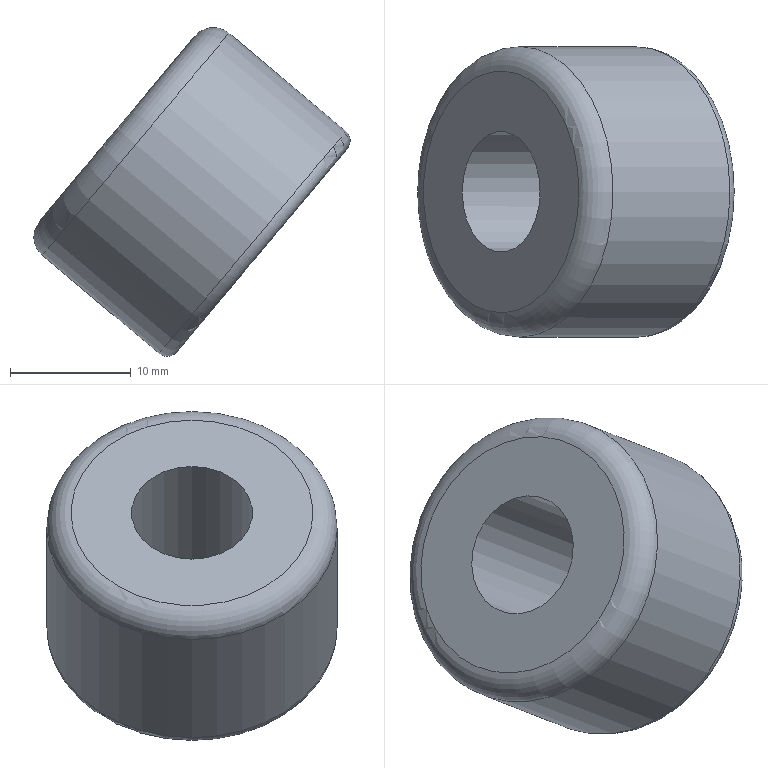Component | NX | BASEBUSHING1_2 | 1 solid | 6 faces | box 26.17 x 24 x 27.2 mm | volume 5761 mm3 | cylinder 2 | plane 2 | torus 2 | commonest cylinder face diameters 24 x1 10 x1
STEP:
#1=CARTESIAN_POINT('',(0.,0.,0.));
#2=DIRECTION('',(0.,0.,1.));
#3=DIRECTION('',(1.,0.,0.));
#4=AXIS2_PLACEMENT_3D('',#1,#2,#3);
#5=CARTESIAN_POINT('',(429.187,0.,-30.182));
#6=VERTEX_POINT('',#5);
#7=CARTESIAN_POINT('',(421.473,0.,-39.375));
#8=DIRECTION('',(0.766,0.,-0.6428));
#9=DIRECTION('',(0.6428,0.,0.766));
#10=AXIS2_PLACEMENT_3D('',#7,#8,#9);
#11=CIRCLE('',#10,12.);
#12=CARTESIAN_POINT('',(431.907,0.,-48.13));
#13=DIRECTION('',(-0.766,0.,0.6428));
#14=DIRECTION('',(0.6428,0.,0.766));
#15=AXIS2_PLACEMENT_3D('',#12,#13,#14);
#16=CYLINDRICAL_SURFACE('',#15,12.);
#17=CARTESIAN_POINT('',(6.283,13.62));
#18=DIRECTION('',(-1.,0.));
#19=VECTOR('',#18,1.);
#20=LINE('',#17,#19);
#21=(GEOMETRIC_REPRESENTATION_CONTEXT(2)PARAMETRIC_REPRESENTATION_CONTEXT()REPRESENTATION_CONTEXT('',''));
#22=DEFINITIONAL_REPRESENTATION('',(#20),#21);
#23=PCURVE('',#16,#22);
#24=CARTESIAN_POINT('',(421.473,0.,-39.375));
#25=DIRECTION('',(-0.766,0.,0.6428));
#26=DIRECTION('',(0.6428,0.,0.766));
#27=AXIS2_PLACEMENT_3D('',#24,#25,#26);
#28=TOROIDAL_SURFACE('',#27,10.,2.);
#29=CARTESIAN_POINT('',(6.283,6.283));
#30=DIRECTION('',(-1.,0.));
#31=VECTOR('',#30,1.);
#32=LINE('',#29,#31);
#33=(GEOMETRIC_REPRESENTATION_CONTEXT(2)PARAMETRIC_REPRESENTATION_CONTEXT()REPRESENTATION_CONTEXT('',''));
#34=DEFINITIONAL_REPRESENTATION('',(#32),#33);
#35=PCURVE('',#28,#34);
#36=SURFACE_CURVE('',#11,(#23,#35),.PCURVE_S1.);
#37=EDGE_CURVE('',#6,#6,#36,.T.);
#38=ORIENTED_EDGE('',*,*,#37,.T.);
#39=CARTESIAN_POINT('',(438.854,0.,-38.295));
#40=VERTEX_POINT('',#39);
#41=CARTESIAN_POINT('',(438.854,-0.,-38.295));
#42=CARTESIAN_POINT('',(429.187,-0.,-30.182));
#43=B_SPLINE_CURVE_WITH_KNOTS('',1,(#41,#42),.UNSPECIFIED.,.F.,.F.,(2,2),(1.,13.62),.PIECEWISE_BEZIER_KNOTS.);
#44=CARTESIAN_POINT('',(0.,0.));
#45=DIRECTION('',(0.,1.));
#46=VECTOR('',#45,1.);
#47=LINE('',#44,#46);
#48=(GEOMETRIC_REPRESENTATION_CONTEXT(2)PARAMETRIC_REPRESENTATION_CONTEXT()REPRESENTATION_CONTEXT('',''));
#49=DEFINITIONAL_REPRESENTATION('',(#47),#48);
#50=PCURVE('',#16,#49);
#51=CARTESIAN_POINT('',(6.283,0.));
#52=DIRECTION('',(0.,1.));
#53=VECTOR('',#52,1.);
#54=LINE('',#51,#53);
#55=(GEOMETRIC_REPRESENTATION_CONTEXT(2)PARAMETRIC_REPRESENTATION_CONTEXT()REPRESENTATION_CONTEXT('',''));
#56=DEFINITIONAL_REPRESENTATION('',(#54),#55);
#57=PCURVE('',#16,#56);
#58=SEAM_CURVE('',#43,(#50,#57),.PCURVE_S1.);
#59=EDGE_CURVE('',#40,#6,#58,.T.);
#60=ORIENTED_EDGE('',*,*,#59,.F.);
#61=CARTESIAN_POINT('',(431.141,0.,-47.487));
#62=DIRECTION('',(-0.766,0.,0.6428));
#63=DIRECTION('',(0.6428,0.,0.766));
#64=AXIS2_PLACEMENT_3D('',#61,#62,#63);
#65=CIRCLE('',#64,12.);
#66=CARTESIAN_POINT('',(0.,1.));
#67=DIRECTION('',(1.,0.));
#68=VECTOR('',#67,1.);
#69=LINE('',#66,#68);
#70=(GEOMETRIC_REPRESENTATION_CONTEXT(2)PARAMETRIC_REPRESENTATION_CONTEXT()REPRESENTATION_CONTEXT('',''));
#71=DEFINITIONAL_REPRESENTATION('',(#69),#70);
#72=PCURVE('',#16,#71);
#73=CARTESIAN_POINT('',(431.141,0.,-47.487));
#74=DIRECTION('',(-0.766,0.,0.6428));
#75=DIRECTION('',(0.6428,0.,0.766));
#76=AXIS2_PLACEMENT_3D('',#73,#74,#75);
#77=TOROIDAL_SURFACE('',#76,11.,1.);
#78=CARTESIAN_POINT('',(0.,6.283));
#79=DIRECTION('',(1.,0.));
#80=VECTOR('',#79,1.);
#81=LINE('',#78,#80);
#82=(GEOMETRIC_REPRESENTATION_CONTEXT(2)PARAMETRIC_REPRESENTATION_CONTEXT()REPRESENTATION_CONTEXT('',''));
#83=DEFINITIONAL_REPRESENTATION('',(#81),#82);
#84=PCURVE('',#77,#83);
#85=SURFACE_CURVE('',#65,(#72,#84),.PCURVE_S1.);
#86=EDGE_CURVE('',#40,#40,#85,.T.);
#87=ORIENTED_EDGE('',*,*,#86,.T.);
#88=ORIENTED_EDGE('',*,*,#59,.T.);
#89=EDGE_LOOP('',(#38,#60,#87,#88));
#90=FACE_BOUND('',#89,.T.);
#91=ADVANCED_FACE('',(#90),#16,.T.);
#92=CARTESIAN_POINT('',(435.121,0.,-44.3));
#93=VERTEX_POINT('',#92);
#94=CARTESIAN_POINT('',(431.907,0.,-48.13));
#95=DIRECTION('',(-0.766,0.,0.6428));
#96=DIRECTION('',(0.6428,0.,0.766));
#97=AXIS2_PLACEMENT_3D('',#94,#95,#96);
#98=CIRCLE('',#97,5.);
#99=CARTESIAN_POINT('',(431.907,0.,-48.13));
#100=DIRECTION('',(-0.766,0.,0.6428));
#101=DIRECTION('',(0.6428,0.,0.766));
#102=AXIS2_PLACEMENT_3D('',#99,#100,#101);
#103=PLANE('',#102);
#104=CARTESIAN_POINT('',(0.,0.));
#105=DIRECTION('',(1.,0.));
#106=AXIS2_PLACEMENT_2D('',#104,#105);
#107=CIRCLE('',#106,5.);
#108=(GEOMETRIC_REPRESENTATION_CONTEXT(2)PARAMETRIC_REPRESENTATION_CONTEXT()REPRESENTATION_CONTEXT('',''));
#109=DEFINITIONAL_REPRESENTATION('',(#107),#108);
#110=PCURVE('',#103,#109);
#111=CARTESIAN_POINT('',(431.907,0.,-48.13));
#112=DIRECTION('',(-0.766,0.,0.6428));
#113=DIRECTION('',(0.6428,0.,0.766));
#114=AXIS2_PLACEMENT_3D('',#111,#112,#113);
#115=CYLINDRICAL_SURFACE('',#114,5.);
#116=CARTESIAN_POINT('',(0.,0.));
#117=DIRECTION('',(1.,0.));
#118=VECTOR('',#117,1.);
#119=LINE('',#116,#118);
#120=(GEOMETRIC_REPRESENTATION_CONTEXT(2)PARAMETRIC_REPRESENTATION_CONTEXT()REPRESENTATION_CONTEXT('',''));
#121=DEFINITIONAL_REPRESENTATION('',(#119),#120);
#122=PCURVE('',#115,#121);
#123=SURFACE_CURVE('',#98,(#110,#122),.PCURVE_S1.);
#124=EDGE_CURVE('',#93,#93,#123,.T.);
#125=ORIENTED_EDGE('',*,*,#124,.T.);
#126=EDGE_LOOP('',(#125));
#127=FACE_BOUND('',#126,.T.);
#128=CARTESIAN_POINT('',(438.978,0.,-39.703));
#129=VERTEX_POINT('',#128);
#130=CARTESIAN_POINT('',(431.907,0.,-48.13));
#131=DIRECTION('',(0.766,0.,-0.6428));
#132=DIRECTION('',(0.6428,0.,0.766));
#133=AXIS2_PLACEMENT_3D('',#130,#131,#132);
#134=CIRCLE('',#133,11.);
#135=CARTESIAN_POINT('',(11.,0.));
#136=CARTESIAN_POINT('',(11.,-19.053));
#137=CARTESIAN_POINT('',(-5.5,-9.526));
#138=CARTESIAN_POINT('',(-22.,-0.));
#139=CARTESIAN_POINT('',(-5.5,9.526));
#140=CARTESIAN_POINT('',(11.,19.053));
#141=CARTESIAN_POINT('',(11.,0.));
#142=(BOUNDED_CURVE()B_SPLINE_CURVE(2,(#135,#136,#137,#138,#139,#140,#141),.UNSPECIFIED.,.T.,.F.)B_SPLINE_CURVE_WITH_KNOTS((1,2,2,2,2,1),(-2.094,0.,2.094,4.189,6.283,8.378),.UNSPECIFIED.)CURVE()GEOMETRIC_REPRESENTATION_ITEM()RATIONAL_B_SPLINE_CURVE((1.,0.5,1.,0.5,1.,0.5,1.))REPRESENTATION_ITEM(''));
#143=(GEOMETRIC_REPRESENTATION_CONTEXT(2)PARAMETRIC_REPRESENTATION_CONTEXT()REPRESENTATION_CONTEXT('',''));
#144=DEFINITIONAL_REPRESENTATION('',(#142),#143);
#145=PCURVE('',#103,#144);
#146=CARTESIAN_POINT('',(6.283,4.712));
#147=DIRECTION('',(-1.,0.));
#148=VECTOR('',#147,1.);
#149=LINE('',#146,#148);
#150=(GEOMETRIC_REPRESENTATION_CONTEXT(2)PARAMETRIC_REPRESENTATION_CONTEXT()REPRESENTATION_CONTEXT('',''));
#151=DEFINITIONAL_REPRESENTATION('',(#149),#150);
#152=PCURVE('',#77,#151);
#153=SURFACE_CURVE('',#134,(#145,#152),.PCURVE_S1.);
#154=EDGE_CURVE('',#129,#129,#153,.T.);
#155=ORIENTED_EDGE('',*,*,#154,.T.);
#156=EDGE_LOOP('',(#155));
#157=FACE_BOUND('',#156,.T.);
#158=ADVANCED_FACE('',(#127,#157),#103,.F.);
#159=CARTESIAN_POINT('',(423.155,0.,-34.259));
#160=VERTEX_POINT('',#159);
#161=CARTESIAN_POINT('',(419.941,0.,-38.089));
#162=DIRECTION('',(-0.766,0.,0.6428));
#163=DIRECTION('',(0.6428,0.,0.766));
#164=AXIS2_PLACEMENT_3D('',#161,#162,#163);
#165=CIRCLE('',#164,5.);
#166=CARTESIAN_POINT('',(419.941,0.,-38.089));
#167=DIRECTION('',(-0.766,0.,0.6428));
#168=DIRECTION('',(0.6428,0.,0.766));
#169=AXIS2_PLACEMENT_3D('',#166,#167,#168);
#170=PLANE('',#169);
#171=CARTESIAN_POINT('',(-0.,0.));
#172=DIRECTION('',(1.,0.));
#173=AXIS2_PLACEMENT_2D('',#171,#172);
#174=CIRCLE('',#173,5.);
#175=(GEOMETRIC_REPRESENTATION_CONTEXT(2)PARAMETRIC_REPRESENTATION_CONTEXT()REPRESENTATION_CONTEXT('',''));
#176=DEFINITIONAL_REPRESENTATION('',(#174),#175);
#177=PCURVE('',#170,#176);
#178=CARTESIAN_POINT('',(0.,15.62));
#179=DIRECTION('',(1.,0.));
#180=VECTOR('',#179,1.);
#181=LINE('',#178,#180);
#182=(GEOMETRIC_REPRESENTATION_CONTEXT(2)PARAMETRIC_REPRESENTATION_CONTEXT()REPRESENTATION_CONTEXT('',''));
#183=DEFINITIONAL_REPRESENTATION('',(#181),#182);
#184=PCURVE('',#115,#183);
#185=SURFACE_CURVE('',#165,(#177,#184),.PCURVE_S1.);
#186=EDGE_CURVE('',#160,#160,#185,.T.);
#187=ORIENTED_EDGE('',*,*,#186,.F.);
#188=EDGE_LOOP('',(#187));
#189=FACE_BOUND('',#188,.T.);
#190=CARTESIAN_POINT('',(426.369,0.,-30.429));
#191=VERTEX_POINT('',#190);
#192=CARTESIAN_POINT('',(419.941,0.,-38.089));
#193=DIRECTION('',(-0.766,0.,0.6428));
#194=DIRECTION('',(0.6428,0.,0.766));
#195=AXIS2_PLACEMENT_3D('',#192,#193,#194);
#196=CIRCLE('',#195,10.);
#197=CARTESIAN_POINT('',(0.,0.));
#198=DIRECTION('',(1.,0.));
#199=AXIS2_PLACEMENT_2D('',#197,#198);
#200=CIRCLE('',#199,10.);
#201=(GEOMETRIC_REPRESENTATION_CONTEXT(2)PARAMETRIC_REPRESENTATION_CONTEXT()REPRESENTATION_CONTEXT('',''));
#202=DEFINITIONAL_REPRESENTATION('',(#200),#201);
#203=PCURVE('',#170,#202);
#204=CARTESIAN_POINT('',(0.,7.854));
#205=DIRECTION('',(1.,0.));
#206=VECTOR('',#205,1.);
#207=LINE('',#204,#206);
#208=(GEOMETRIC_REPRESENTATION_CONTEXT(2)PARAMETRIC_REPRESENTATION_CONTEXT()REPRESENTATION_CONTEXT('',''));
#209=DEFINITIONAL_REPRESENTATION('',(#207),#208);
#210=PCURVE('',#28,#209);
#211=SURFACE_CURVE('',#196,(#203,#210),.PCURVE_S1.);
#212=EDGE_CURVE('',#191,#191,#211,.T.);
#213=ORIENTED_EDGE('',*,*,#212,.T.);
#214=EDGE_LOOP('',(#213));
#215=FACE_BOUND('',#214,.T.);
#216=ADVANCED_FACE('',(#189,#215),#170,.T.);
#217=ORIENTED_EDGE('',*,*,#37,.F.);
#218=CARTESIAN_POINT('',(429.187,0.,-30.182));
#219=CARTESIAN_POINT('',(428.777,0.,-29.839));
#220=CARTESIAN_POINT('',(428.269,0.,-29.634));
#221=CARTESIAN_POINT('',(427.716,0.,-29.596));
#222=CARTESIAN_POINT('',(427.178,0.,-29.73));
#223=CARTESIAN_POINT('',(426.713,0.,-30.019));
#224=CARTESIAN_POINT('',(426.369,0.,-30.429));
#225=(BOUNDED_CURVE()B_SPLINE_CURVE(6,(#218,#219,#220,#221,#222,#223,#224),.UNSPECIFIED.,.F.,.F.)B_SPLINE_CURVE_WITH_KNOTS((7,7),(0.,1.571),.PIECEWISE_BEZIER_KNOTS.)CURVE()GEOMETRIC_REPRESENTATION_ITEM()RATIONAL_B_SPLINE_CURVE((1.031,1.01,0.9979,0.994,0.9979,1.01,1.031))REPRESENTATION_ITEM(''));
#226=CARTESIAN_POINT('',(6.283,6.283));
#227=DIRECTION('',(0.,1.));
#228=VECTOR('',#227,1.);
#229=LINE('',#226,#228);
#230=(GEOMETRIC_REPRESENTATION_CONTEXT(2)PARAMETRIC_REPRESENTATION_CONTEXT()REPRESENTATION_CONTEXT('',''));
#231=DEFINITIONAL_REPRESENTATION('',(#229),#230);
#232=PCURVE('',#28,#231);
#233=CARTESIAN_POINT('',(0.,6.283));
#234=DIRECTION('',(0.,1.));
#235=VECTOR('',#234,1.);
#236=LINE('',#233,#235);
#237=(GEOMETRIC_REPRESENTATION_CONTEXT(2)PARAMETRIC_REPRESENTATION_CONTEXT()REPRESENTATION_CONTEXT('',''));
#238=DEFINITIONAL_REPRESENTATION('',(#236),#237);
#239=PCURVE('',#28,#238);
#240=SEAM_CURVE('',#225,(#232,#239),.PCURVE_S1.);
#241=EDGE_CURVE('',#6,#191,#240,.T.);
#242=ORIENTED_EDGE('',*,*,#241,.T.);
#243=ORIENTED_EDGE('',*,*,#212,.F.);
#244=ORIENTED_EDGE('',*,*,#241,.F.);
#245=EDGE_LOOP('',(#217,#242,#243,#244));
#246=FACE_BOUND('',#245,.T.);
#247=ADVANCED_FACE('',(#246),#28,.T.);
#248=ORIENTED_EDGE('',*,*,#154,.F.);
#249=CARTESIAN_POINT('',(438.978,0.,-39.703));
#250=CARTESIAN_POINT('',(439.15,0.,-39.499));
#251=CARTESIAN_POINT('',(439.252,0.,-39.244));
#252=CARTESIAN_POINT('',(439.271,0.,-38.968));
#253=CARTESIAN_POINT('',(439.204,0.,-38.699));
#254=CARTESIAN_POINT('',(439.059,0.,-38.466));
#255=CARTESIAN_POINT('',(438.854,0.,-38.295));
#256=(BOUNDED_CURVE()B_SPLINE_CURVE(6,(#249,#250,#251,#252,#253,#254,#255),.UNSPECIFIED.,.F.,.F.)B_SPLINE_CURVE_WITH_KNOTS((7,7),(4.712,6.283),.PIECEWISE_BEZIER_KNOTS.)CURVE()GEOMETRIC_REPRESENTATION_ITEM()RATIONAL_B_SPLINE_CURVE((1.031,1.01,0.9979,0.994,0.9979,1.01,1.031))REPRESENTATION_ITEM(''));
#257=CARTESIAN_POINT('',(6.283,0.));
#258=DIRECTION('',(0.,1.));
#259=VECTOR('',#258,1.);
#260=LINE('',#257,#259);
#261=(GEOMETRIC_REPRESENTATION_CONTEXT(2)PARAMETRIC_REPRESENTATION_CONTEXT()REPRESENTATION_CONTEXT('',''));
#262=DEFINITIONAL_REPRESENTATION('',(#260),#261);
#263=PCURVE('',#77,#262);
#264=CARTESIAN_POINT('',(0.,0.));
#265=DIRECTION('',(0.,1.));
#266=VECTOR('',#265,1.);
#267=LINE('',#264,#266);
#268=(GEOMETRIC_REPRESENTATION_CONTEXT(2)PARAMETRIC_REPRESENTATION_CONTEXT()REPRESENTATION_CONTEXT('',''));
#269=DEFINITIONAL_REPRESENTATION('',(#267),#268);
#270=PCURVE('',#77,#269);
#271=SEAM_CURVE('',#256,(#263,#270),.PCURVE_S1.);
#272=EDGE_CURVE('',#129,#40,#271,.T.);
#273=ORIENTED_EDGE('',*,*,#272,.T.);
#274=ORIENTED_EDGE('',*,*,#86,.F.);
#275=ORIENTED_EDGE('',*,*,#272,.F.);
#276=EDGE_LOOP('',(#248,#273,#274,#275));
#277=FACE_BOUND('',#276,.T.);
#278=ADVANCED_FACE('',(#277),#77,.T.);
#279=ORIENTED_EDGE('',*,*,#186,.F.);
#280=CARTESIAN_POINT('',(435.121,-0.,-44.3));
#281=CARTESIAN_POINT('',(423.155,-0.,-34.259));
#282=B_SPLINE_CURVE_WITH_KNOTS('',1,(#280,#281),.UNSPECIFIED.,.F.,.F.,(2,2),(0.,15.62),.PIECEWISE_BEZIER_KNOTS.);
#283=CARTESIAN_POINT('',(0.,0.));
#284=DIRECTION('',(0.,1.));
#285=VECTOR('',#284,1.);
#286=LINE('',#283,#285);
#287=(GEOMETRIC_REPRESENTATION_CONTEXT(2)PARAMETRIC_REPRESENTATION_CONTEXT()REPRESENTATION_CONTEXT('',''));
#288=DEFINITIONAL_REPRESENTATION('',(#286),#287);
#289=PCURVE('',#115,#288);
#290=CARTESIAN_POINT('',(6.283,0.));
#291=DIRECTION('',(0.,1.));
#292=VECTOR('',#291,1.);
#293=LINE('',#290,#292);
#294=(GEOMETRIC_REPRESENTATION_CONTEXT(2)PARAMETRIC_REPRESENTATION_CONTEXT()REPRESENTATION_CONTEXT('',''));
#295=DEFINITIONAL_REPRESENTATION('',(#293),#294);
#296=PCURVE('',#115,#295);
#297=SEAM_CURVE('',#282,(#289,#296),.PCURVE_S1.);
#298=EDGE_CURVE('',#93,#160,#297,.T.);
#299=ORIENTED_EDGE('',*,*,#298,.F.);
#300=ORIENTED_EDGE('',*,*,#124,.T.);
#301=ORIENTED_EDGE('',*,*,#298,.T.);
#302=EDGE_LOOP('',(#279,#299,#300,#301));
#303=FACE_BOUND('',#302,.F.);
#304=ADVANCED_FACE('',(#303),#115,.F.);
#305=CLOSED_SHELL('',(#91,#158,#216,#247,#278,#304));
#306=MANIFOLD_SOLID_BREP('',#305);
#307=(LENGTH_UNIT()NAMED_UNIT(*)SI_UNIT(.MILLI.,.METRE.));
#308=UNCERTAINTY_MEASURE_WITH_UNIT(LENGTH_MEASURE(0.00001),#307,'','');
#309=(NAMED_UNIT(*)PLANE_ANGLE_UNIT()SI_UNIT($,.RADIAN.));
#310=(NAMED_UNIT(*)SI_UNIT($,.STERADIAN.)SOLID_ANGLE_UNIT());
#311=(GEOMETRIC_REPRESENTATION_CONTEXT(3)GLOBAL_UNCERTAINTY_ASSIGNED_CONTEXT((#308))GLOBAL_UNIT_ASSIGNED_CONTEXT((#307,#309,#310))REPRESENTATION_CONTEXT('',''));
#312=ADVANCED_BREP_SHAPE_REPRESENTATION('',(#4,#306),#311);